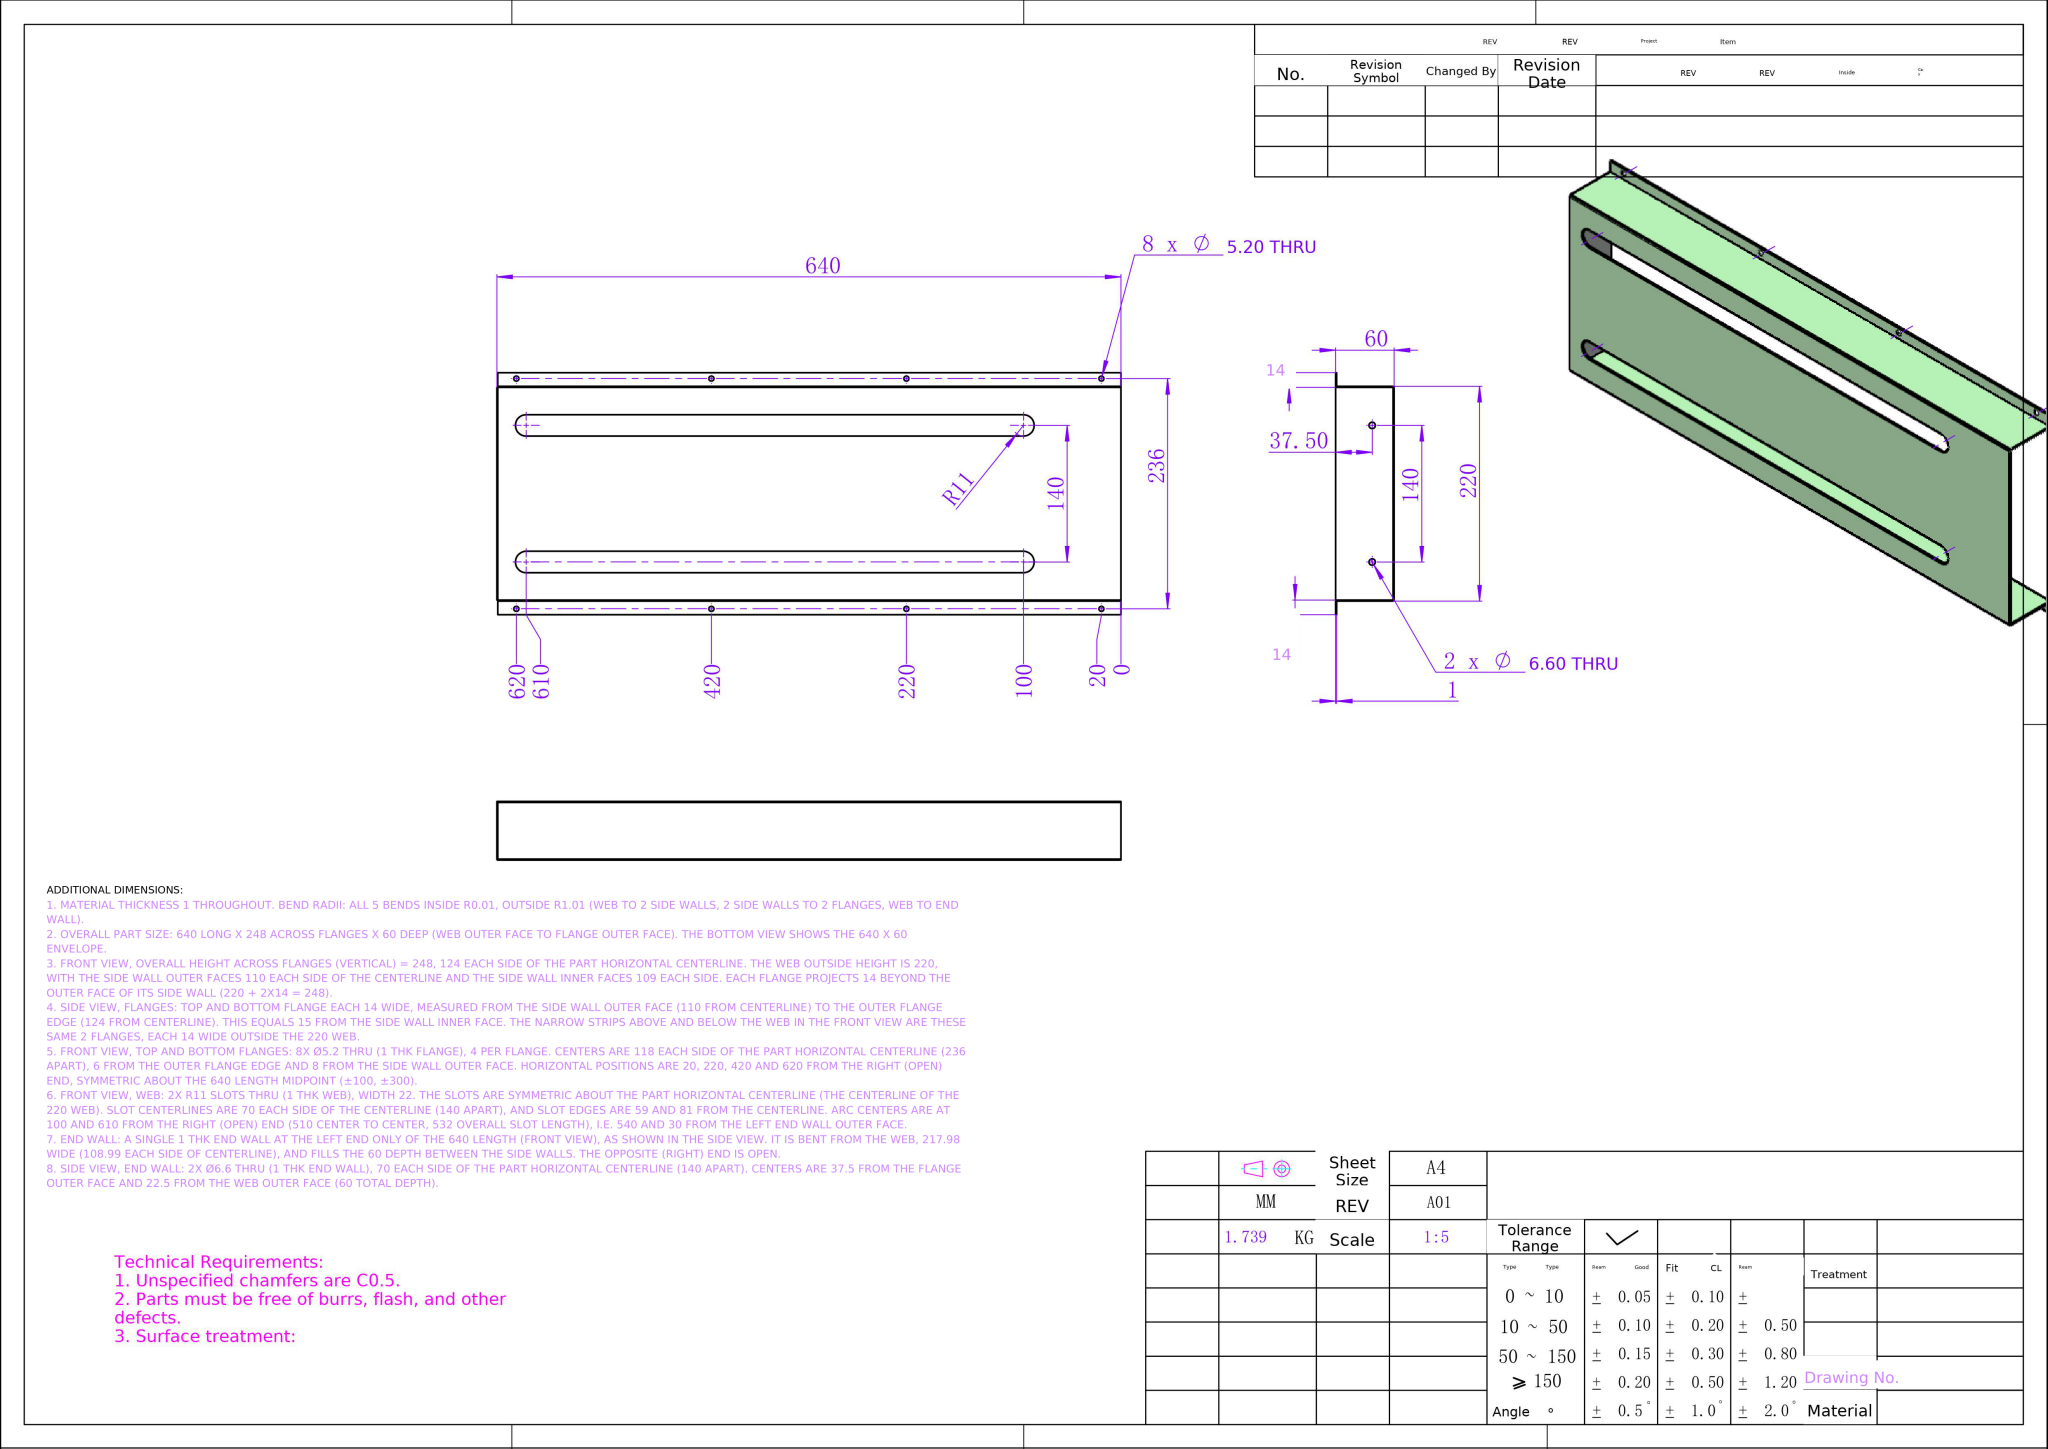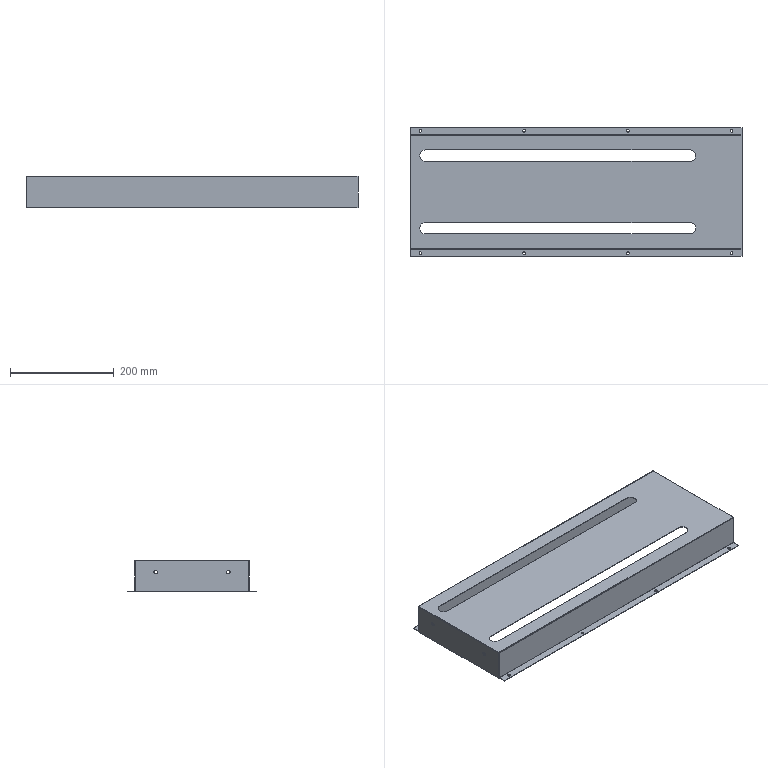Part | NX | mm | 1 solid | 76 faces | box 640 x 248 x 60 mm | volume 222906 mm3 | cylinder 36 | plane 36 | spline 4 | commonest cylinder face diameters 5.2 x16 22 x6 2.02 x5 0.02 x5 6.6 x4